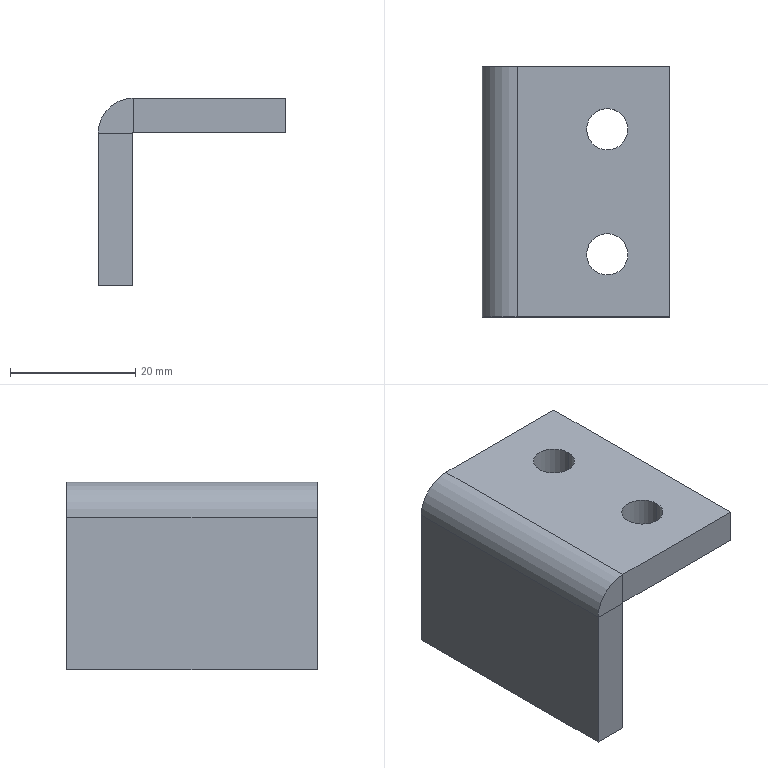Component | SolidWorks | StopA-0510-1 | 1 solid | 18 faces | box 30 x 40 x 30 mm | volume 11345 mm3 | plane 12 | cylinder 6 | commonest cylinder face diameters 6.6 x4 11.2 x1 0.2 x1 | material Q235-A
STEP:
#1=CARTESIAN_POINT('',(-34.98,-0.3783,139.469));
#2=VERTEX_POINT('',#1);
#3=CARTESIAN_POINT('',(-34.72,-0.3783,139.469));
#4=VERTEX_POINT('',#3);
#5=CARTESIAN_POINT('',(-34.85,-0.3783,139.469));
#6=DIRECTION('',(0.,-0.,-1.));
#7=DIRECTION('',(1.,0.,0.));
#8=AXIS2_PLACEMENT_3D('',#5,#6,#7);
#9=CIRCLE('',#8,0.1299);
#10=EDGE_CURVE('',#2,#4,#9,.T.);
#11=ORIENTED_EDGE('',*,*,#10,.F.);
#12=CARTESIAN_POINT('',(-34.98,-0.3783,139.252));
#13=VERTEX_POINT('',#12);
#14=CARTESIAN_POINT('',(-34.98,-0.3783,139.252));
#15=DIRECTION('',(0.,-0.,-1.));
#16=VECTOR('',#15,39.37);
#17=LINE('',#14,#16);
#18=EDGE_CURVE('',#2,#13,#17,.T.);
#19=ORIENTED_EDGE('',*,*,#18,.T.);
#20=CARTESIAN_POINT('',(-34.72,-0.3783,139.252));
#21=VERTEX_POINT('',#20);
#22=CARTESIAN_POINT('',(-34.85,-0.3783,139.252));
#23=DIRECTION('',(0.,-0.,-1.));
#24=DIRECTION('',(1.,0.,0.));
#25=AXIS2_PLACEMENT_3D('',#22,#23,#24);
#26=CIRCLE('',#25,0.1299);
#27=EDGE_CURVE('',#13,#21,#26,.T.);
#28=ORIENTED_EDGE('',*,*,#27,.T.);
#29=CARTESIAN_POINT('',(-34.72,-0.3783,139.252));
#30=DIRECTION('',(0.,-0.,-1.));
#31=VECTOR('',#30,39.37);
#32=LINE('',#29,#31);
#33=EDGE_CURVE('',#4,#21,#32,.T.);
#34=ORIENTED_EDGE('',*,*,#33,.F.);
#35=EDGE_LOOP('',(#11,#19,#28,#34));
#36=FACE_OUTER_BOUND('',#35,.T.);
#37=CARTESIAN_POINT('',(-34.85,-0.3783,139.252));
#38=DIRECTION('',(0.,-0.,-1.));
#39=DIRECTION('',(1.,0.,0.));
#40=AXIS2_PLACEMENT_3D('',#37,#38,#39);
#41=CYLINDRICAL_SURFACE('',#40,0.1299);
#42=ADVANCED_FACE('',(#36),#41,.F.);
#43=CARTESIAN_POINT('',(-34.98,0.4091,139.469));
#44=VERTEX_POINT('',#43);
#45=CARTESIAN_POINT('',(-34.72,0.4091,139.469));
#46=VERTEX_POINT('',#45);
#47=CARTESIAN_POINT('',(-34.85,0.4091,139.469));
#48=DIRECTION('',(0.,-0.,-1.));
#49=DIRECTION('',(1.,0.,0.));
#50=AXIS2_PLACEMENT_3D('',#47,#48,#49);
#51=CIRCLE('',#50,0.1299);
#52=EDGE_CURVE('',#44,#46,#51,.T.);
#53=ORIENTED_EDGE('',*,*,#52,.F.);
#54=CARTESIAN_POINT('',(-34.98,0.4091,139.252));
#55=VERTEX_POINT('',#54);
#56=CARTESIAN_POINT('',(-34.98,0.4091,139.252));
#57=DIRECTION('',(0.,-0.,-1.));
#58=VECTOR('',#57,39.37);
#59=LINE('',#56,#58);
#60=EDGE_CURVE('',#44,#55,#59,.T.);
#61=ORIENTED_EDGE('',*,*,#60,.T.);
#62=CARTESIAN_POINT('',(-34.72,0.4091,139.252));
#63=VERTEX_POINT('',#62);
#64=CARTESIAN_POINT('',(-34.85,0.4091,139.252));
#65=DIRECTION('',(0.,-0.,-1.));
#66=DIRECTION('',(1.,0.,0.));
#67=AXIS2_PLACEMENT_3D('',#64,#65,#66);
#68=CIRCLE('',#67,0.1299);
#69=EDGE_CURVE('',#55,#63,#68,.T.);
#70=ORIENTED_EDGE('',*,*,#69,.T.);
#71=CARTESIAN_POINT('',(-34.72,0.4091,139.252));
#72=DIRECTION('',(0.,-0.,-1.));
#73=VECTOR('',#72,39.37);
#74=LINE('',#71,#73);
#75=EDGE_CURVE('',#46,#63,#74,.T.);
#76=ORIENTED_EDGE('',*,*,#75,.F.);
#77=EDGE_LOOP('',(#53,#61,#70,#76));
#78=FACE_OUTER_BOUND('',#77,.T.);
#79=CARTESIAN_POINT('',(-34.85,0.4091,139.252));
#80=DIRECTION('',(0.,-0.,-1.));
#81=DIRECTION('',(1.,0.,0.));
#82=AXIS2_PLACEMENT_3D('',#79,#80,#81);
#83=CYLINDRICAL_SURFACE('',#82,0.1299);
#84=ADVANCED_FACE('',(#78),#83,.F.);
#85=CARTESIAN_POINT('',(-35.417,-0.772,139.469));
#86=VERTEX_POINT('',#85);
#87=CARTESIAN_POINT('',(-35.417,-0.772,139.252));
#88=VERTEX_POINT('',#87);
#89=CARTESIAN_POINT('',(-35.417,-0.772,139.469));
#90=DIRECTION('',(0.,-0.,-1.));
#91=VECTOR('',#90,39.37);
#92=LINE('',#89,#91);
#93=EDGE_CURVE('',#86,#88,#92,.T.);
#94=ORIENTED_EDGE('',*,*,#93,.F.);
#95=CARTESIAN_POINT('',(-35.638,-0.772,139.248));
#96=VERTEX_POINT('',#95);
#97=CARTESIAN_POINT('',(-35.417,-0.772,139.248));
#98=DIRECTION('',(-0.,1.,-0.));
#99=DIRECTION('',(1.,0.,0.));
#100=AXIS2_PLACEMENT_3D('',#97,#98,#99);
#101=CIRCLE('',#100,0.2205);
#102=EDGE_CURVE('',#96,#86,#101,.T.);
#103=ORIENTED_EDGE('',*,*,#102,.F.);
#104=CARTESIAN_POINT('',(-35.421,-0.772,139.248));
#105=VERTEX_POINT('',#104);
#106=CARTESIAN_POINT('',(-35.421,-0.772,139.248));
#107=DIRECTION('',(-1.,-0.,-0.));
#108=VECTOR('',#107,39.37);
#109=LINE('',#106,#108);
#110=EDGE_CURVE('',#105,#96,#109,.T.);
#111=ORIENTED_EDGE('',*,*,#110,.F.);
#112=CARTESIAN_POINT('',(-35.417,-0.772,139.248));
#113=DIRECTION('',(-0.,1.,-0.));
#114=DIRECTION('',(1.,0.,0.));
#115=AXIS2_PLACEMENT_3D('',#112,#113,#114);
#116=CIRCLE('',#115,0.003937);
#117=EDGE_CURVE('',#105,#88,#116,.T.);
#118=ORIENTED_EDGE('',*,*,#117,.T.);
#119=EDGE_LOOP('',(#94,#103,#111,#118));
#120=FACE_OUTER_BOUND('',#119,.T.);
#121=CARTESIAN_POINT('',(-35.417,-0.772,139.469));
#122=DIRECTION('',(0.,-1.,0.));
#123=DIRECTION('',(1.,0.,0.));
#124=AXIS2_PLACEMENT_3D('',#121,#122,#123);
#125=PLANE('',#124);
#126=ADVANCED_FACE('',(#120),#125,.T.);
#127=CARTESIAN_POINT('',(-34.457,-0.772,139.469));
#128=VERTEX_POINT('',#127);
#129=CARTESIAN_POINT('',(-35.638,-0.772,139.469));
#130=DIRECTION('',(1.,0.,0.));
#131=VECTOR('',#130,39.37);
#132=LINE('',#129,#131);
#133=EDGE_CURVE('',#86,#128,#132,.T.);
#134=ORIENTED_EDGE('',*,*,#133,.F.);
#135=ORIENTED_EDGE('',*,*,#93,.T.);
#136=CARTESIAN_POINT('',(-34.457,-0.772,139.252));
#137=VERTEX_POINT('',#136);
#138=CARTESIAN_POINT('',(-35.638,-0.772,139.252));
#139=DIRECTION('',(1.,0.,0.));
#140=VECTOR('',#139,39.37);
#141=LINE('',#138,#140);
#142=EDGE_CURVE('',#88,#137,#141,.T.);
#143=ORIENTED_EDGE('',*,*,#142,.T.);
#144=CARTESIAN_POINT('',(-34.457,-0.772,139.469));
#145=DIRECTION('',(0.,-0.,-1.));
#146=VECTOR('',#145,39.37);
#147=LINE('',#144,#146);
#148=EDGE_CURVE('',#128,#137,#147,.T.);
#149=ORIENTED_EDGE('',*,*,#148,.F.);
#150=EDGE_LOOP('',(#134,#135,#143,#149));
#151=FACE_OUTER_BOUND('',#150,.T.);
#152=CARTESIAN_POINT('',(-35.421,-0.772,139.248));
#153=DIRECTION('',(0.,-1.,0.));
#154=DIRECTION('',(1.,0.,0.));
#155=AXIS2_PLACEMENT_3D('',#152,#153,#154);
#156=PLANE('',#155);
#157=ADVANCED_FACE('',(#151),#156,.T.);
#158=CARTESIAN_POINT('',(-35.638,0.8028,139.248));
#159=VERTEX_POINT('',#158);
#160=CARTESIAN_POINT('',(-35.421,0.8028,139.248));
#161=VERTEX_POINT('',#160);
#162=CARTESIAN_POINT('',(-35.638,0.8028,139.248));
#163=DIRECTION('',(1.,0.,0.));
#164=VECTOR('',#163,39.37);
#165=LINE('',#162,#164);
#166=EDGE_CURVE('',#159,#161,#165,.T.);
#167=ORIENTED_EDGE('',*,*,#166,.F.);
#168=CARTESIAN_POINT('',(-35.417,0.8028,139.469));
#169=VERTEX_POINT('',#168);
#170=CARTESIAN_POINT('',(-35.417,0.8028,139.248));
#171=DIRECTION('',(-0.,1.,-0.));
#172=DIRECTION('',(1.,0.,0.));
#173=AXIS2_PLACEMENT_3D('',#170,#171,#172);
#174=CIRCLE('',#173,0.2205);
#175=EDGE_CURVE('',#159,#169,#174,.T.);
#176=ORIENTED_EDGE('',*,*,#175,.T.);
#177=CARTESIAN_POINT('',(-35.417,0.8028,139.252));
#178=VERTEX_POINT('',#177);
#179=CARTESIAN_POINT('',(-35.417,0.8028,139.252));
#180=DIRECTION('',(-0.,0.,1.));
#181=VECTOR('',#180,39.37);
#182=LINE('',#179,#181);
#183=EDGE_CURVE('',#178,#169,#182,.T.);
#184=ORIENTED_EDGE('',*,*,#183,.F.);
#185=CARTESIAN_POINT('',(-35.417,0.8028,139.248));
#186=DIRECTION('',(-0.,1.,-0.));
#187=DIRECTION('',(1.,0.,0.));
#188=AXIS2_PLACEMENT_3D('',#185,#186,#187);
#189=CIRCLE('',#188,0.003937);
#190=EDGE_CURVE('',#161,#178,#189,.T.);
#191=ORIENTED_EDGE('',*,*,#190,.F.);
#192=EDGE_LOOP('',(#167,#176,#184,#191));
#193=FACE_OUTER_BOUND('',#192,.T.);
#194=CARTESIAN_POINT('',(-35.638,0.8028,139.248));
#195=DIRECTION('',(-0.,1.,-0.));
#196=DIRECTION('',(-1.,-0.,-0.));
#197=AXIS2_PLACEMENT_3D('',#194,#195,#196);
#198=PLANE('',#197);
#199=ADVANCED_FACE('',(#193),#198,.T.);
#200=CARTESIAN_POINT('',(-35.638,0.8028,138.287));
#201=VERTEX_POINT('',#200);
#202=CARTESIAN_POINT('',(-35.638,0.8028,138.287));
#203=DIRECTION('',(-0.,0.,1.));
#204=VECTOR('',#203,39.37);
#205=LINE('',#202,#204);
#206=EDGE_CURVE('',#201,#159,#205,.T.);
#207=ORIENTED_EDGE('',*,*,#206,.T.);
#208=ORIENTED_EDGE('',*,*,#166,.T.);
#209=CARTESIAN_POINT('',(-35.421,0.8028,138.287));
#210=VERTEX_POINT('',#209);
#211=CARTESIAN_POINT('',(-35.421,0.8028,138.287));
#212=DIRECTION('',(-0.,0.,1.));
#213=VECTOR('',#212,39.37);
#214=LINE('',#211,#213);
#215=EDGE_CURVE('',#210,#161,#214,.T.);
#216=ORIENTED_EDGE('',*,*,#215,.F.);
#217=CARTESIAN_POINT('',(-35.421,0.8028,138.287));
#218=DIRECTION('',(-1.,-0.,-0.));
#219=VECTOR('',#218,39.37);
#220=LINE('',#217,#219);
#221=EDGE_CURVE('',#210,#201,#220,.T.);
#222=ORIENTED_EDGE('',*,*,#221,.T.);
#223=EDGE_LOOP('',(#207,#208,#216,#222));
#224=FACE_OUTER_BOUND('',#223,.T.);
#225=CARTESIAN_POINT('',(-35.417,0.8028,139.252));
#226=DIRECTION('',(-0.,1.,-0.));
#227=DIRECTION('',(-1.,-0.,-0.));
#228=AXIS2_PLACEMENT_3D('',#225,#226,#227);
#229=PLANE('',#228);
#230=ADVANCED_FACE('',(#224),#229,.T.);
#231=CARTESIAN_POINT('',(-34.85,-0.3783,139.252));
#232=DIRECTION('',(0.,-0.,-1.));
#233=DIRECTION('',(1.,0.,0.));
#234=AXIS2_PLACEMENT_3D('',#231,#232,#233);
#235=CIRCLE('',#234,0.1299);
#236=EDGE_CURVE('',#21,#13,#235,.T.);
#237=ORIENTED_EDGE('',*,*,#236,.F.);
#238=ORIENTED_EDGE('',*,*,#27,.F.);
#239=EDGE_LOOP('',(#237,#238));
#240=FACE_BOUND('',#239,.T.);
#241=CARTESIAN_POINT('',(-34.85,0.4091,139.252));
#242=DIRECTION('',(0.,-0.,-1.));
#243=DIRECTION('',(1.,0.,0.));
#244=AXIS2_PLACEMENT_3D('',#241,#242,#243);
#245=CIRCLE('',#244,0.1299);
#246=EDGE_CURVE('',#63,#55,#245,.T.);
#247=ORIENTED_EDGE('',*,*,#246,.F.);
#248=ORIENTED_EDGE('',*,*,#69,.F.);
#249=EDGE_LOOP('',(#247,#248));
#250=FACE_BOUND('',#249,.T.);
#251=CARTESIAN_POINT('',(-34.457,0.8028,139.252));
#252=VERTEX_POINT('',#251);
#253=CARTESIAN_POINT('',(-35.638,0.8028,139.252));
#254=DIRECTION('',(1.,0.,0.));
#255=VECTOR('',#254,39.37);
#256=LINE('',#253,#255);
#257=EDGE_CURVE('',#178,#252,#256,.T.);
#258=ORIENTED_EDGE('',*,*,#257,.T.);
#259=CARTESIAN_POINT('',(-34.457,-0.772,139.252));
#260=DIRECTION('',(-0.,1.,-0.));
#261=VECTOR('',#260,39.37);
#262=LINE('',#259,#261);
#263=EDGE_CURVE('',#137,#252,#262,.T.);
#264=ORIENTED_EDGE('',*,*,#263,.F.);
#265=ORIENTED_EDGE('',*,*,#142,.F.);
#266=CARTESIAN_POINT('',(-35.417,-0.772,139.252));
#267=DIRECTION('',(-0.,1.,-0.));
#268=VECTOR('',#267,39.37);
#269=LINE('',#266,#268);
#270=EDGE_CURVE('',#88,#178,#269,.T.);
#271=ORIENTED_EDGE('',*,*,#270,.T.);
#272=EDGE_LOOP('',(#258,#264,#265,#271));
#273=FACE_OUTER_BOUND('',#272,.T.);
#274=CARTESIAN_POINT('',(-35.638,-0.772,139.252));
#275=DIRECTION('',(-0.,0.,1.));
#276=DIRECTION('',(-1.,-0.,-0.));
#277=AXIS2_PLACEMENT_3D('',#274,#275,#276);
#278=PLANE('',#277);
#279=ADVANCED_FACE('',(#240,#250,#273),#278,.F.);
#280=CARTESIAN_POINT('',(-34.457,0.8028,139.469));
#281=VERTEX_POINT('',#280);
#282=CARTESIAN_POINT('',(-34.457,0.8028,139.469));
#283=DIRECTION('',(0.,-0.,-1.));
#284=VECTOR('',#283,39.37);
#285=LINE('',#282,#284);
#286=EDGE_CURVE('',#281,#252,#285,.T.);
#287=ORIENTED_EDGE('',*,*,#286,.F.);
#288=CARTESIAN_POINT('',(-34.457,-0.772,139.469));
#289=DIRECTION('',(-0.,1.,-0.));
#290=VECTOR('',#289,39.37);
#291=LINE('',#288,#290);
#292=EDGE_CURVE('',#128,#281,#291,.T.);
#293=ORIENTED_EDGE('',*,*,#292,.F.);
#294=ORIENTED_EDGE('',*,*,#148,.T.);
#295=ORIENTED_EDGE('',*,*,#263,.T.);
#296=EDGE_LOOP('',(#287,#293,#294,#295));
#297=FACE_OUTER_BOUND('',#296,.T.);
#298=CARTESIAN_POINT('',(-34.457,-0.772,139.469));
#299=DIRECTION('',(1.,0.,0.));
#300=DIRECTION('',(-0.,1.,-0.));
#301=AXIS2_PLACEMENT_3D('',#298,#299,#300);
#302=PLANE('',#301);
#303=ADVANCED_FACE('',(#297),#302,.T.);
#304=CARTESIAN_POINT('',(-34.85,-0.3783,139.469));
#305=DIRECTION('',(0.,-0.,-1.));
#306=DIRECTION('',(1.,0.,0.));
#307=AXIS2_PLACEMENT_3D('',#304,#305,#306);
#308=CIRCLE('',#307,0.1299);
#309=EDGE_CURVE('',#4,#2,#308,.T.);
#310=ORIENTED_EDGE('',*,*,#309,.T.);
#311=ORIENTED_EDGE('',*,*,#10,.T.);
#312=EDGE_LOOP('',(#310,#311));
#313=FACE_BOUND('',#312,.T.);
#314=CARTESIAN_POINT('',(-34.85,0.4091,139.469));
#315=DIRECTION('',(0.,-0.,-1.));
#316=DIRECTION('',(1.,0.,0.));
#317=AXIS2_PLACEMENT_3D('',#314,#315,#316);
#318=CIRCLE('',#317,0.1299);
#319=EDGE_CURVE('',#46,#44,#318,.T.);
#320=ORIENTED_EDGE('',*,*,#319,.T.);
#321=ORIENTED_EDGE('',*,*,#52,.T.);
#322=EDGE_LOOP('',(#320,#321));
#323=FACE_BOUND('',#322,.T.);
#324=CARTESIAN_POINT('',(-35.638,0.8028,139.469));
#325=DIRECTION('',(1.,0.,0.));
#326=VECTOR('',#325,39.37);
#327=LINE('',#324,#326);
#328=EDGE_CURVE('',#169,#281,#327,.T.);
#329=ORIENTED_EDGE('',*,*,#328,.F.);
#330=CARTESIAN_POINT('',(-35.417,-0.772,139.469));
#331=DIRECTION('',(-0.,1.,-0.));
#332=VECTOR('',#331,39.37);
#333=LINE('',#330,#332);
#334=EDGE_CURVE('',#86,#169,#333,.T.);
#335=ORIENTED_EDGE('',*,*,#334,.F.);
#336=ORIENTED_EDGE('',*,*,#133,.T.);
#337=ORIENTED_EDGE('',*,*,#292,.T.);
#338=EDGE_LOOP('',(#329,#335,#336,#337));
#339=FACE_OUTER_BOUND('',#338,.T.);
#340=CARTESIAN_POINT('',(-35.638,-0.772,139.469));
#341=DIRECTION('',(-0.,0.,1.));
#342=DIRECTION('',(-1.,-0.,-0.));
#343=AXIS2_PLACEMENT_3D('',#340,#341,#342);
#344=PLANE('',#343);
#345=ADVANCED_FACE('',(#313,#323,#339),#344,.T.);
#346=ORIENTED_EDGE('',*,*,#175,.F.);
#347=CARTESIAN_POINT('',(-35.638,-0.772,139.248));
#348=DIRECTION('',(-0.,1.,-0.));
#349=VECTOR('',#348,39.37);
#350=LINE('',#347,#349);
#351=EDGE_CURVE('',#96,#159,#350,.T.);
#352=ORIENTED_EDGE('',*,*,#351,.F.);
#353=ORIENTED_EDGE('',*,*,#102,.T.);
#354=ORIENTED_EDGE('',*,*,#334,.T.);
#355=EDGE_LOOP('',(#346,#352,#353,#354));
#356=FACE_OUTER_BOUND('',#355,.T.);
#357=CARTESIAN_POINT('',(-35.417,-0.772,139.248));
#358=DIRECTION('',(-0.,1.,-0.));
#359=DIRECTION('',(-1.,0.,0.));
#360=AXIS2_PLACEMENT_3D('',#357,#358,#359);
#361=CYLINDRICAL_SURFACE('',#360,0.2205);
#362=ADVANCED_FACE('',(#356),#361,.T.);
#363=ORIENTED_EDGE('',*,*,#206,.F.);
#364=CARTESIAN_POINT('',(-35.638,-0.772,138.287));
#365=VERTEX_POINT('',#364);
#366=CARTESIAN_POINT('',(-35.638,-0.772,138.287));
#367=DIRECTION('',(-0.,1.,-0.));
#368=VECTOR('',#367,39.37);
#369=LINE('',#366,#368);
#370=EDGE_CURVE('',#365,#201,#369,.T.);
#371=ORIENTED_EDGE('',*,*,#370,.F.);
#372=CARTESIAN_POINT('',(-35.638,-0.772,138.287));
#373=DIRECTION('',(-0.,0.,1.));
#374=VECTOR('',#373,39.37);
#375=LINE('',#372,#374);
#376=EDGE_CURVE('',#365,#96,#375,.T.);
#377=ORIENTED_EDGE('',*,*,#376,.T.);
#378=ORIENTED_EDGE('',*,*,#351,.T.);
#379=EDGE_LOOP('',(#363,#371,#377,#378));
#380=FACE_OUTER_BOUND('',#379,.T.);
#381=CARTESIAN_POINT('',(-35.638,-0.772,138.287));
#382=DIRECTION('',(-1.,-0.,-0.));
#383=DIRECTION('',(0.,-1.,0.));
#384=AXIS2_PLACEMENT_3D('',#381,#382,#383);
#385=PLANE('',#384);
#386=ADVANCED_FACE('',(#380),#385,.T.);
#387=ORIENTED_EDGE('',*,*,#221,.F.);
#388=CARTESIAN_POINT('',(-35.421,-0.772,138.287));
#389=VERTEX_POINT('',#388);
#390=CARTESIAN_POINT('',(-35.421,-0.772,138.287));
#391=DIRECTION('',(-0.,1.,-0.));
#392=VECTOR('',#391,39.37);
#393=LINE('',#390,#392);
#394=EDGE_CURVE('',#389,#210,#393,.T.);
#395=ORIENTED_EDGE('',*,*,#394,.F.);
#396=CARTESIAN_POINT('',(-35.421,-0.772,138.287));
#397=DIRECTION('',(-1.,-0.,-0.));
#398=VECTOR('',#397,39.37);
#399=LINE('',#396,#398);
#400=EDGE_CURVE('',#389,#365,#399,.T.);
#401=ORIENTED_EDGE('',*,*,#400,.T.);
#402=ORIENTED_EDGE('',*,*,#370,.T.);
#403=EDGE_LOOP('',(#387,#395,#401,#402));
#404=FACE_OUTER_BOUND('',#403,.T.);
#405=CARTESIAN_POINT('',(-35.421,-0.772,138.287));
#406=DIRECTION('',(0.,-0.,-1.));
#407=DIRECTION('',(1.,0.,0.));
#408=AXIS2_PLACEMENT_3D('',#405,#406,#407);
#409=PLANE('',#408);
#410=ADVANCED_FACE('',(#404),#409,.T.);
#411=ORIENTED_EDGE('',*,*,#215,.T.);
#412=CARTESIAN_POINT('',(-35.421,-0.772,139.248));
#413=DIRECTION('',(-0.,1.,-0.));
#414=VECTOR('',#413,39.37);
#415=LINE('',#412,#414);
#416=EDGE_CURVE('',#105,#161,#415,.T.);
#417=ORIENTED_EDGE('',*,*,#416,.F.);
#418=CARTESIAN_POINT('',(-35.421,-0.772,138.287));
#419=DIRECTION('',(-0.,0.,1.));
#420=VECTOR('',#419,39.37);
#421=LINE('',#418,#420);
#422=EDGE_CURVE('',#389,#105,#421,.T.);
#423=ORIENTED_EDGE('',*,*,#422,.F.);
#424=ORIENTED_EDGE('',*,*,#394,.T.);
#425=EDGE_LOOP('',(#411,#417,#423,#424));
#426=FACE_OUTER_BOUND('',#425,.T.);
#427=CARTESIAN_POINT('',(-35.421,-0.772,138.287));
#428=DIRECTION('',(-1.,-0.,-0.));
#429=DIRECTION('',(0.,-1.,0.));
#430=AXIS2_PLACEMENT_3D('',#427,#428,#429);
#431=PLANE('',#430);
#432=ADVANCED_FACE('',(#426),#431,.F.);
#433=ORIENTED_EDGE('',*,*,#190,.T.);
#434=ORIENTED_EDGE('',*,*,#270,.F.);
#435=ORIENTED_EDGE('',*,*,#117,.F.);
#436=ORIENTED_EDGE('',*,*,#416,.T.);
#437=EDGE_LOOP('',(#433,#434,#435,#436));
#438=FACE_OUTER_BOUND('',#437,.T.);
#439=CARTESIAN_POINT('',(-35.417,-0.772,139.248));
#440=DIRECTION('',(-0.,1.,-0.));
#441=DIRECTION('',(-1.,0.,0.));
#442=AXIS2_PLACEMENT_3D('',#439,#440,#441);
#443=CYLINDRICAL_SURFACE('',#442,0.003937);
#444=ADVANCED_FACE('',(#438),#443,.F.);
#445=ORIENTED_EDGE('',*,*,#422,.T.);
#446=ORIENTED_EDGE('',*,*,#110,.T.);
#447=ORIENTED_EDGE('',*,*,#376,.F.);
#448=ORIENTED_EDGE('',*,*,#400,.F.);
#449=EDGE_LOOP('',(#445,#446,#447,#448));
#450=FACE_OUTER_BOUND('',#449,.T.);
#451=CARTESIAN_POINT('',(-35.417,-0.772,139.248));
#452=DIRECTION('',(0.,-1.,0.));
#453=DIRECTION('',(1.,0.,0.));
#454=AXIS2_PLACEMENT_3D('',#451,#452,#453);
#455=PLANE('',#454);
#456=ADVANCED_FACE('',(#450),#455,.T.);
#457=ORIENTED_EDGE('',*,*,#257,.F.);
#458=ORIENTED_EDGE('',*,*,#183,.T.);
#459=ORIENTED_EDGE('',*,*,#328,.T.);
#460=ORIENTED_EDGE('',*,*,#286,.T.);
#461=EDGE_LOOP('',(#457,#458,#459,#460));
#462=FACE_OUTER_BOUND('',#461,.T.);
#463=CARTESIAN_POINT('',(-35.417,0.8028,139.248));
#464=DIRECTION('',(0.,-1.,0.));
#465=DIRECTION('',(1.,0.,0.));
#466=AXIS2_PLACEMENT_3D('',#463,#464,#465);
#467=PLANE('',#466);
#468=ADVANCED_FACE('',(#462),#467,.F.);
#469=ORIENTED_EDGE('',*,*,#60,.F.);
#470=ORIENTED_EDGE('',*,*,#319,.F.);
#471=ORIENTED_EDGE('',*,*,#75,.T.);
#472=ORIENTED_EDGE('',*,*,#246,.T.);
#473=EDGE_LOOP('',(#469,#470,#471,#472));
#474=FACE_OUTER_BOUND('',#473,.T.);
#475=CARTESIAN_POINT('',(-34.85,0.4091,139.252));
#476=DIRECTION('',(0.,-0.,-1.));
#477=DIRECTION('',(1.,0.,0.));
#478=AXIS2_PLACEMENT_3D('',#475,#476,#477);
#479=CYLINDRICAL_SURFACE('',#478,0.1299);
#480=ADVANCED_FACE('',(#474),#479,.F.);
#481=ORIENTED_EDGE('',*,*,#18,.F.);
#482=ORIENTED_EDGE('',*,*,#309,.F.);
#483=ORIENTED_EDGE('',*,*,#33,.T.);
#484=ORIENTED_EDGE('',*,*,#236,.T.);
#485=EDGE_LOOP('',(#481,#482,#483,#484));
#486=FACE_OUTER_BOUND('',#485,.T.);
#487=CARTESIAN_POINT('',(-34.85,-0.3783,139.252));
#488=DIRECTION('',(0.,-0.,-1.));
#489=DIRECTION('',(1.,0.,0.));
#490=AXIS2_PLACEMENT_3D('',#487,#488,#489);
#491=CYLINDRICAL_SURFACE('',#490,0.1299);
#492=ADVANCED_FACE('',(#486),#491,.F.);
#493=CLOSED_SHELL('',(#42,#84,#126,#157,#199,#230,#279,#303,#345,#362,#386,#410,#432,#444,#456,#468,#480,#492));
#494=MANIFOLD_SOLID_BREP('',#493);
#495=CARTESIAN_POINT('',(0.,0.,0.));
#496=DIRECTION('',(0.,0.,1.));
#497=DIRECTION('',(1.,0.,0.));
#498=AXIS2_PLACEMENT_3D('',#495,#496,#497);
#499=(LENGTH_UNIT()NAMED_UNIT(*)SI_UNIT($,.METRE.));
#500=LENGTH_MEASURE_WITH_UNIT(LENGTH_MEASURE(0.0254),#499);
#501=DIMENSIONAL_EXPONENTS(1.,0.,0.,0.,0.,0.,0.);
#502=(CONVERSION_BASED_UNIT('',#500)LENGTH_UNIT()NAMED_UNIT(#501));
#503=UNCERTAINTY_MEASURE_WITH_UNIT(LENGTH_MEASURE(0.00001),#502,'','');
#504=(NAMED_UNIT(*)PLANE_ANGLE_UNIT()SI_UNIT($,.RADIAN.));
#505=(NAMED_UNIT(*)SI_UNIT($,.STERADIAN.)SOLID_ANGLE_UNIT());
#506=(GEOMETRIC_REPRESENTATION_CONTEXT(3)GLOBAL_UNCERTAINTY_ASSIGNED_CONTEXT((#503))GLOBAL_UNIT_ASSIGNED_CONTEXT((#502,#504,#505))REPRESENTATION_CONTEXT('',''));
#507=ADVANCED_BREP_SHAPE_REPRESENTATION('',(#494,#498),#506);
#508=COLOUR_RGB('',0.7922,0.8196,0.9333);
#509=FILL_AREA_STYLE_COLOUR('',#508);
#510=FILL_AREA_STYLE('',(#509));
#511=SURFACE_STYLE_FILL_AREA(#510);
#512=SURFACE_SIDE_STYLE('',(#511));
#513=SURFACE_STYLE_USAGE(.BOTH.,#512);
#514=PRESENTATION_STYLE_ASSIGNMENT((#513));
#515=STYLED_ITEM('',(#514),#494);
#516=PRESENTATION_LAYER_ASSIGNMENT('','',(#515));
#517=(LENGTH_UNIT()NAMED_UNIT(*)SI_UNIT($,.METRE.));
#518=LENGTH_MEASURE_WITH_UNIT(LENGTH_MEASURE(0.0254),#517);
#519=DIMENSIONAL_EXPONENTS(1.,0.,0.,0.,0.,0.,0.);
#520=(CONVERSION_BASED_UNIT('',#518)LENGTH_UNIT()NAMED_UNIT(#519));
#521=UNCERTAINTY_MEASURE_WITH_UNIT(LENGTH_MEASURE(0.00001),#520,'','');
#522=(NAMED_UNIT(*)PLANE_ANGLE_UNIT()SI_UNIT($,.RADIAN.));
#523=(NAMED_UNIT(*)SI_UNIT($,.STERADIAN.)SOLID_ANGLE_UNIT());
#524=(GEOMETRIC_REPRESENTATION_CONTEXT(3)GLOBAL_UNCERTAINTY_ASSIGNED_CONTEXT((#521))GLOBAL_UNIT_ASSIGNED_CONTEXT((#520,#522,#523))REPRESENTATION_CONTEXT('',''));
#525=MECHANICAL_DESIGN_GEOMETRIC_PRESENTATION_REPRESENTATION('',(#515),#524);